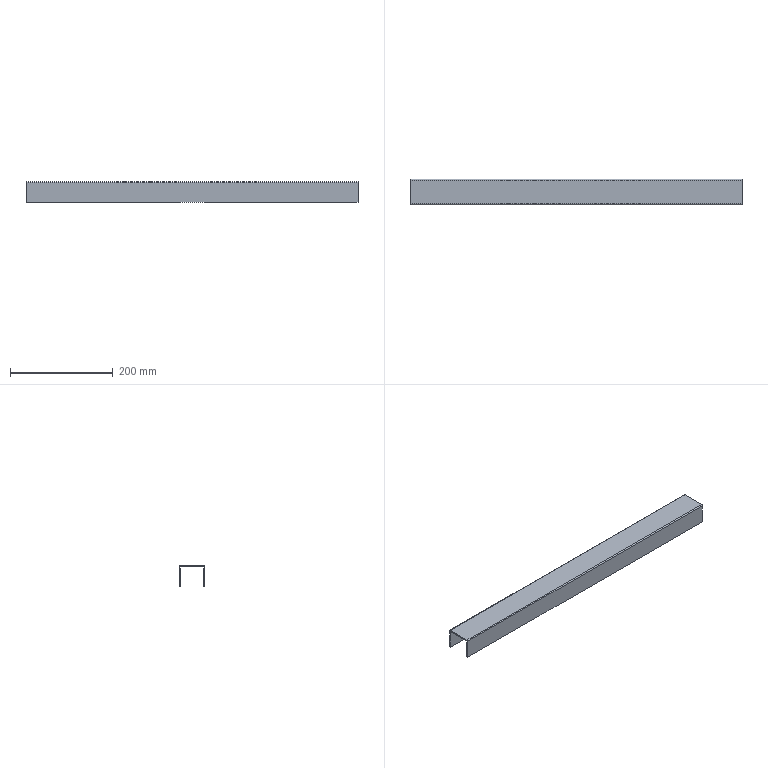Component | SolidWorks | FrameAssembly-1_FrameWeldment-1_LowerBendPlate-1 | 1 solid | 24 faces | box 645 x 50 x 40 mm | volume 195847 mm3 | plane 18 | cylinder 6 | commonest cylinder face diameters 9 x4 4 x2
build123d program:
from build123d import *

# Parameters (mm, degrees)
BOSS_EXTRUDE1_DEPTH = 645
SKETCH6_W           = 37.5
SKETCH6_H           = 45
CUT_EXTRUDE1_DEPTH  = 649.171
CUT_EXTRUDE2_REACH  = 330.795
SKETCH7_W           = 30
SKETCH7_H           = 50
CUT_EXTRUDE3_DEPTH  = 329.424
CUT_EXTRUDE4_REACH  = 330.795


with BuildPart() as part:
    # Sketch5 → Boss-Extrude1 (new body)
    with BuildSketch(Plane(origin=(0, 0, -322.5), x_dir=(-1, 0, 0), z_dir=(0, 0, -1))):
        with BuildLine():
            Line((-40, 50), (-40, 0))
            Line((-40, 0), (-2, 0))
            ThreePointArc((-2, 0), (-0.5858, 0.5858), (0, 2))
            Line((0, 2), (0, 48))
            ThreePointArc((0, 48), (-0.5858, 49.414), (-2, 50))
            Line((-2, 50), (-40, 50))
        make_face()
    extrude(amount=-BOSS_EXTRUDE1_DEPTH)

    # Sketch6 → Cut-Extrude1 (cut, through all)
    with BuildSketch(Plane.XY.offset(322.5)):
        with Locations((21.25, 25)):
            Rectangle(SKETCH6_W, SKETCH6_H)
    extrude(amount=-CUT_EXTRUDE1_DEPTH, mode=Mode.SUBTRACT)

    # Sketch7 → Cut-Extrude2 (cut, up to next)
    with BuildSketch(Plane.XZ, mode=Mode.PRIVATE) as cut_extrude2_sk1:
        with Locations((25, 0)):
            Rectangle(SKETCH7_W, SKETCH7_H)
    cut_extrude2_tool1 = extrude(cut_extrude2_sk1.sketch, amount=-CUT_EXTRUDE2_REACH, mode=Mode.PRIVATE) & part.part
    add(cut_extrude2_tool1.solids().sort_by_distance((25, 0, 0))[0], mode=Mode.SUBTRACT)

    # Sketch8 → Cut-Extrude3 (cut, through all)
    with BuildSketch(Plane(origin=(0, 2.5, 0), x_dir=(-1, 0, 0), z_dir=(0, 1, 0))):
        with BuildLine():
            Line((-26, -247.5), (-14, -247.5))
            ThreePointArc((-14, -247.5), (-9.5, -243), (-14, -238.5))
            Line((-14, -238.5), (-26, -238.5))
            ThreePointArc((-26, -238.5), (-30.5, -243), (-26, -247.5))
        make_face()
    extrude(amount=-CUT_EXTRUDE3_DEPTH, mode=Mode.SUBTRACT)

    # Sketch9 → Cut-Extrude4 (cut, up to next)
    with BuildSketch(Plane.XZ, mode=Mode.PRIVATE) as cut_extrude4_sk1:
        with BuildLine():
            Line((26, 247.5), (14, 247.5))
            ThreePointArc((14, 247.5), (9.5, 243), (14, 238.5))
            Line((14, 238.5), (26, 238.5))
            ThreePointArc((26, 238.5), (30.5, 243), (26, 247.5))
        make_face()
    cut_extrude4_tool1 = extrude(cut_extrude4_sk1.sketch, amount=-CUT_EXTRUDE4_REACH, mode=Mode.PRIVATE) & part.part
    add(cut_extrude4_tool1.solids().sort_by_distance((20, 0, 243))[0], mode=Mode.SUBTRACT)


solid = part.part

# Placed as in the assembly
solid = solid.moved(Location((-298.746, -158.627, -16.5), (180, -90, 0)))
STEP:
#1=COLOUR_RGB('',0.7922,0.8196,0.9333);
#2=FILL_AREA_STYLE_COLOUR('',#1);
#3=FILL_AREA_STYLE('',(#2));
#4=SURFACE_STYLE_FILL_AREA(#3);
#5=SURFACE_SIDE_STYLE('',(#4));
#6=SURFACE_STYLE_USAGE(.BOTH.,#5);
#7=PRESENTATION_STYLE_ASSIGNMENT((#6));
#8=CARTESIAN_POINT('',(-10.777,-6.344,-2.224));
#9=VERTEX_POINT('',#8);
#10=CARTESIAN_POINT('',(-10.777,-6.245,-2.224));
#11=VERTEX_POINT('',#10);
#12=CARTESIAN_POINT('',(-10.777,-8.214,-2.224));
#13=DIRECTION('',(0.,1.,0.));
#14=VECTOR('',#13,39.37);
#15=LINE('',#12,#14);
#16=EDGE_CURVE('',#9,#11,#15,.T.);
#17=ORIENTED_EDGE('',*,*,#16,.T.);
#18=CARTESIAN_POINT('',(0.9352,-6.245,-2.224));
#19=VERTEX_POINT('',#18);
#20=CARTESIAN_POINT('',(-24.459,-6.245,-2.224));
#21=DIRECTION('',(1.,0.,-0.));
#22=VECTOR('',#21,39.37);
#23=LINE('',#20,#22);
#24=EDGE_CURVE('',#11,#19,#23,.T.);
#25=ORIENTED_EDGE('',*,*,#24,.T.);
#26=CARTESIAN_POINT('',(0.9352,-6.344,-2.224));
#27=VERTEX_POINT('',#26);
#28=CARTESIAN_POINT('',(0.9352,-8.214,-2.224));
#29=DIRECTION('',(0.,1.,0.));
#30=VECTOR('',#29,39.37);
#31=LINE('',#28,#30);
#32=EDGE_CURVE('',#27,#19,#31,.T.);
#33=ORIENTED_EDGE('',*,*,#32,.F.);
#34=CARTESIAN_POINT('',(0.9352,-6.344,-2.224));
#35=DIRECTION('',(-1.,0.,0.));
#36=VECTOR('',#35,39.37);
#37=LINE('',#34,#36);
#38=EDGE_CURVE('',#27,#9,#37,.T.);
#39=ORIENTED_EDGE('',*,*,#38,.T.);
#40=EDGE_LOOP('',(#17,#25,#33,#39));
#41=FACE_OUTER_BOUND('',#40,.T.);
#42=CARTESIAN_POINT('',(-24.459,-8.214,-2.224));
#43=DIRECTION('',(-0.,0.,-1.));
#44=DIRECTION('',(1.,0.,-0.));
#45=AXIS2_PLACEMENT_3D('',#42,#43,#44);
#46=PLANE('',#45);
#47=ADVANCED_FACE('',(#41),#46,.T.);
#48=CARTESIAN_POINT('',(-12.746,-6.344,-2.224));
#49=VERTEX_POINT('',#48);
#50=CARTESIAN_POINT('',(-12.746,-6.245,-2.224));
#51=VERTEX_POINT('',#50);
#52=CARTESIAN_POINT('',(-12.746,-8.214,-2.224));
#53=DIRECTION('',(0.,1.,0.));
#54=VECTOR('',#53,39.37);
#55=LINE('',#52,#54);
#56=EDGE_CURVE('',#49,#51,#55,.T.);
#57=ORIENTED_EDGE('',*,*,#56,.F.);
#58=CARTESIAN_POINT('',(-24.459,-6.344,-2.224));
#59=VERTEX_POINT('',#58);
#60=CARTESIAN_POINT('',(0.9352,-6.344,-2.224));
#61=DIRECTION('',(-1.,0.,0.));
#62=VECTOR('',#61,39.37);
#63=LINE('',#60,#62);
#64=EDGE_CURVE('',#49,#59,#63,.T.);
#65=ORIENTED_EDGE('',*,*,#64,.T.);
#66=CARTESIAN_POINT('',(-24.459,-6.245,-2.224));
#67=VERTEX_POINT('',#66);
#68=CARTESIAN_POINT('',(-24.459,-8.214,-2.224));
#69=DIRECTION('',(0.,1.,0.));
#70=VECTOR('',#69,39.37);
#71=LINE('',#68,#70);
#72=EDGE_CURVE('',#59,#67,#71,.T.);
#73=ORIENTED_EDGE('',*,*,#72,.T.);
#74=CARTESIAN_POINT('',(-24.459,-6.245,-2.224));
#75=DIRECTION('',(1.,0.,-0.));
#76=VECTOR('',#75,39.37);
#77=LINE('',#74,#76);
#78=EDGE_CURVE('',#67,#51,#77,.T.);
#79=ORIENTED_EDGE('',*,*,#78,.T.);
#80=EDGE_LOOP('',(#57,#65,#73,#79));
#81=FACE_OUTER_BOUND('',#80,.T.);
#82=CARTESIAN_POINT('',(-24.459,-8.214,-2.224));
#83=DIRECTION('',(-0.,0.,-1.));
#84=DIRECTION('',(1.,0.,-0.));
#85=AXIS2_PLACEMENT_3D('',#82,#83,#84);
#86=PLANE('',#85);
#87=ADVANCED_FACE('',(#81),#86,.T.);
#88=CARTESIAN_POINT('',(0.9352,-8.214,-0.7283));
#89=VERTEX_POINT('',#88);
#90=CARTESIAN_POINT('',(0.9352,-8.214,-2.224));
#91=VERTEX_POINT('',#90);
#92=CARTESIAN_POINT('',(0.9352,-8.214,-0.7283));
#93=DIRECTION('',(-0.,0.,-1.));
#94=VECTOR('',#93,39.37);
#95=LINE('',#92,#94);
#96=EDGE_CURVE('',#89,#91,#95,.T.);
#97=ORIENTED_EDGE('',*,*,#96,.F.);
#98=CARTESIAN_POINT('',(-24.459,-8.214,-0.7283));
#99=VERTEX_POINT('',#98);
#100=CARTESIAN_POINT('',(-24.459,-8.214,-0.7283));
#101=DIRECTION('',(1.,0.,-0.));
#102=VECTOR('',#101,39.37);
#103=LINE('',#100,#102);
#104=EDGE_CURVE('',#99,#89,#103,.T.);
#105=ORIENTED_EDGE('',*,*,#104,.F.);
#106=CARTESIAN_POINT('',(-24.459,-8.214,-2.224));
#107=VERTEX_POINT('',#106);
#108=CARTESIAN_POINT('',(-24.459,-8.214,-0.7283));
#109=DIRECTION('',(-0.,0.,-1.));
#110=VECTOR('',#109,39.37);
#111=LINE('',#108,#110);
#112=EDGE_CURVE('',#99,#107,#111,.T.);
#113=ORIENTED_EDGE('',*,*,#112,.T.);
#114=CARTESIAN_POINT('',(-24.459,-8.214,-2.224));
#115=DIRECTION('',(1.,0.,-0.));
#116=VECTOR('',#115,39.37);
#117=LINE('',#114,#116);
#118=EDGE_CURVE('',#107,#91,#117,.T.);
#119=ORIENTED_EDGE('',*,*,#118,.T.);
#120=EDGE_LOOP('',(#97,#105,#113,#119));
#121=FACE_OUTER_BOUND('',#120,.T.);
#122=CARTESIAN_POINT('',(-24.459,-8.214,-0.7283));
#123=DIRECTION('',(0.,-1.,0.));
#124=DIRECTION('',(-1.,0.,0.));
#125=AXIS2_PLACEMENT_3D('',#122,#123,#124);
#126=PLANE('',#125);
#127=ADVANCED_FACE('',(#121),#126,.T.);
#128=CARTESIAN_POINT('',(0.9352,-8.135,-0.6496));
#129=VERTEX_POINT('',#128);
#130=CARTESIAN_POINT('',(0.9352,-8.135,-0.7283));
#131=DIRECTION('',(1.,0.,-0.));
#132=DIRECTION('',(0.,0.,1.));
#133=AXIS2_PLACEMENT_3D('',#130,#131,#132);
#134=CIRCLE('',#133,0.07874);
#135=EDGE_CURVE('',#129,#89,#134,.T.);
#136=ORIENTED_EDGE('',*,*,#135,.F.);
#137=CARTESIAN_POINT('',(-24.459,-8.135,-0.6496));
#138=VERTEX_POINT('',#137);
#139=CARTESIAN_POINT('',(-24.459,-8.135,-0.6496));
#140=DIRECTION('',(1.,0.,-0.));
#141=VECTOR('',#140,39.37);
#142=LINE('',#139,#141);
#143=EDGE_CURVE('',#138,#129,#142,.T.);
#144=ORIENTED_EDGE('',*,*,#143,.F.);
#145=CARTESIAN_POINT('',(-24.459,-8.135,-0.7283));
#146=DIRECTION('',(1.,0.,-0.));
#147=DIRECTION('',(0.,0.,1.));
#148=AXIS2_PLACEMENT_3D('',#145,#146,#147);
#149=CIRCLE('',#148,0.07874);
#150=EDGE_CURVE('',#138,#99,#149,.T.);
#151=ORIENTED_EDGE('',*,*,#150,.T.);
#152=ORIENTED_EDGE('',*,*,#104,.T.);
#153=EDGE_LOOP('',(#136,#144,#151,#152));
#154=FACE_OUTER_BOUND('',#153,.T.);
#155=CARTESIAN_POINT('',(-24.459,-8.135,-0.7283));
#156=DIRECTION('',(1.,0.,-0.));
#157=DIRECTION('',(0.,0.,1.));
#158=AXIS2_PLACEMENT_3D('',#155,#156,#157);
#159=CYLINDRICAL_SURFACE('',#158,0.07874);
#160=ADVANCED_FACE('',(#154),#159,.T.);
#161=CARTESIAN_POINT('',(0.9352,-6.324,-0.6496));
#162=VERTEX_POINT('',#161);
#163=CARTESIAN_POINT('',(0.9352,-6.324,-0.6496));
#164=DIRECTION('',(0.,-1.,0.));
#165=VECTOR('',#164,39.37);
#166=LINE('',#163,#165);
#167=EDGE_CURVE('',#162,#129,#166,.T.);
#168=ORIENTED_EDGE('',*,*,#167,.F.);
#169=CARTESIAN_POINT('',(-24.459,-6.324,-0.6496));
#170=VERTEX_POINT('',#169);
#171=CARTESIAN_POINT('',(-24.459,-6.324,-0.6496));
#172=DIRECTION('',(1.,0.,-0.));
#173=VECTOR('',#172,39.37);
#174=LINE('',#171,#173);
#175=EDGE_CURVE('',#170,#162,#174,.T.);
#176=ORIENTED_EDGE('',*,*,#175,.F.);
#177=CARTESIAN_POINT('',(-24.459,-6.324,-0.6496));
#178=DIRECTION('',(0.,-1.,0.));
#179=VECTOR('',#178,39.37);
#180=LINE('',#177,#179);
#181=EDGE_CURVE('',#170,#138,#180,.T.);
#182=ORIENTED_EDGE('',*,*,#181,.T.);
#183=ORIENTED_EDGE('',*,*,#143,.T.);
#184=EDGE_LOOP('',(#168,#176,#182,#183));
#185=FACE_OUTER_BOUND('',#184,.T.);
#186=CARTESIAN_POINT('',(-24.459,-6.324,-0.6496));
#187=DIRECTION('',(0.,0.,1.));
#188=DIRECTION('',(-0.,1.,-0.));
#189=AXIS2_PLACEMENT_3D('',#186,#187,#188);
#190=PLANE('',#189);
#191=ADVANCED_FACE('',(#185),#190,.T.);
#192=CARTESIAN_POINT('',(0.9352,-6.245,-0.7283));
#193=VERTEX_POINT('',#192);
#194=CARTESIAN_POINT('',(0.9352,-6.324,-0.7283));
#195=DIRECTION('',(1.,0.,-0.));
#196=DIRECTION('',(0.,0.,1.));
#197=AXIS2_PLACEMENT_3D('',#194,#195,#196);
#198=CIRCLE('',#197,0.07874);
#199=EDGE_CURVE('',#193,#162,#198,.T.);
#200=ORIENTED_EDGE('',*,*,#199,.F.);
#201=CARTESIAN_POINT('',(-24.459,-6.245,-0.7283));
#202=VERTEX_POINT('',#201);
#203=CARTESIAN_POINT('',(-24.459,-6.245,-0.7283));
#204=DIRECTION('',(1.,0.,-0.));
#205=VECTOR('',#204,39.37);
#206=LINE('',#203,#205);
#207=EDGE_CURVE('',#202,#193,#206,.T.);
#208=ORIENTED_EDGE('',*,*,#207,.F.);
#209=CARTESIAN_POINT('',(-24.459,-6.324,-0.7283));
#210=DIRECTION('',(1.,0.,-0.));
#211=DIRECTION('',(0.,0.,1.));
#212=AXIS2_PLACEMENT_3D('',#209,#210,#211);
#213=CIRCLE('',#212,0.07874);
#214=EDGE_CURVE('',#202,#170,#213,.T.);
#215=ORIENTED_EDGE('',*,*,#214,.T.);
#216=ORIENTED_EDGE('',*,*,#175,.T.);
#217=EDGE_LOOP('',(#200,#208,#215,#216));
#218=FACE_OUTER_BOUND('',#217,.T.);
#219=CARTESIAN_POINT('',(-24.459,-6.324,-0.7283));
#220=DIRECTION('',(1.,0.,-0.));
#221=DIRECTION('',(0.,0.,1.));
#222=AXIS2_PLACEMENT_3D('',#219,#220,#221);
#223=CYLINDRICAL_SURFACE('',#222,0.07874);
#224=ADVANCED_FACE('',(#218),#223,.T.);
#225=CARTESIAN_POINT('',(-21.151,-6.245,-1.673));
#226=VERTEX_POINT('',#225);
#227=CARTESIAN_POINT('',(-21.506,-6.245,-1.673));
#228=VERTEX_POINT('',#227);
#229=CARTESIAN_POINT('',(-21.329,-6.245,-1.673));
#230=DIRECTION('',(0.,1.,0.));
#231=DIRECTION('',(1.,0.,0.));
#232=AXIS2_PLACEMENT_3D('',#229,#230,#231);
#233=CIRCLE('',#232,0.1772);
#234=EDGE_CURVE('',#226,#228,#233,.T.);
#235=ORIENTED_EDGE('',*,*,#234,.F.);
#236=CARTESIAN_POINT('',(-21.151,-6.245,-1.201));
#237=VERTEX_POINT('',#236);
#238=CARTESIAN_POINT('',(-21.151,-6.245,-1.201));
#239=DIRECTION('',(0.,0.,-1.));
#240=VECTOR('',#239,39.37);
#241=LINE('',#238,#240);
#242=EDGE_CURVE('',#237,#226,#241,.T.);
#243=ORIENTED_EDGE('',*,*,#242,.F.);
#244=CARTESIAN_POINT('',(-21.506,-6.245,-1.201));
#245=VERTEX_POINT('',#244);
#246=CARTESIAN_POINT('',(-21.329,-6.245,-1.201));
#247=DIRECTION('',(0.,1.,0.));
#248=DIRECTION('',(1.,0.,0.));
#249=AXIS2_PLACEMENT_3D('',#246,#247,#248);
#250=CIRCLE('',#249,0.1772);
#251=EDGE_CURVE('',#245,#237,#250,.T.);
#252=ORIENTED_EDGE('',*,*,#251,.F.);
#253=CARTESIAN_POINT('',(-21.506,-6.245,-1.673));
#254=DIRECTION('',(0.,0.,1.));
#255=VECTOR('',#254,39.37);
#256=LINE('',#253,#255);
#257=EDGE_CURVE('',#228,#245,#256,.T.);
#258=ORIENTED_EDGE('',*,*,#257,.F.);
#259=EDGE_LOOP('',(#235,#243,#252,#258));
#260=FACE_BOUND('',#259,.T.);
#261=CARTESIAN_POINT('',(-2.372,-6.245,-1.673));
#262=VERTEX_POINT('',#261);
#263=CARTESIAN_POINT('',(-2.018,-6.245,-1.673));
#264=VERTEX_POINT('',#263);
#265=CARTESIAN_POINT('',(-2.195,-6.245,-1.673));
#266=DIRECTION('',(0.,-1.,0.));
#267=DIRECTION('',(-1.,0.,0.));
#268=AXIS2_PLACEMENT_3D('',#265,#266,#267);
#269=CIRCLE('',#268,0.1772);
#270=EDGE_CURVE('',#262,#264,#269,.T.);
#271=ORIENTED_EDGE('',*,*,#270,.T.);
#272=CARTESIAN_POINT('',(-2.018,-6.245,-1.201));
#273=VERTEX_POINT('',#272);
#274=CARTESIAN_POINT('',(-2.018,-6.245,-1.673));
#275=DIRECTION('',(0.,0.,1.));
#276=VECTOR('',#275,39.37);
#277=LINE('',#274,#276);
#278=EDGE_CURVE('',#264,#273,#277,.T.);
#279=ORIENTED_EDGE('',*,*,#278,.T.);
#280=CARTESIAN_POINT('',(-2.372,-6.245,-1.201));
#281=VERTEX_POINT('',#280);
#282=CARTESIAN_POINT('',(-2.195,-6.245,-1.201));
#283=DIRECTION('',(0.,-1.,0.));
#284=DIRECTION('',(-1.,0.,0.));
#285=AXIS2_PLACEMENT_3D('',#282,#283,#284);
#286=CIRCLE('',#285,0.1772);
#287=EDGE_CURVE('',#273,#281,#286,.T.);
#288=ORIENTED_EDGE('',*,*,#287,.T.);
#289=CARTESIAN_POINT('',(-2.372,-6.245,-1.201));
#290=DIRECTION('',(-0.,0.,-1.));
#291=VECTOR('',#290,39.37);
#292=LINE('',#289,#291);
#293=EDGE_CURVE('',#281,#262,#292,.T.);
#294=ORIENTED_EDGE('',*,*,#293,.T.);
#295=EDGE_LOOP('',(#271,#279,#288,#294));
#296=FACE_BOUND('',#295,.T.);
#297=CARTESIAN_POINT('',(-10.777,-6.245,-1.043));
#298=VERTEX_POINT('',#297);
#299=CARTESIAN_POINT('',(-10.777,-6.245,-1.043));
#300=DIRECTION('',(-0.,0.,-1.));
#301=VECTOR('',#300,39.37);
#302=LINE('',#299,#301);
#303=EDGE_CURVE('',#298,#11,#302,.T.);
#304=ORIENTED_EDGE('',*,*,#303,.F.);
#305=CARTESIAN_POINT('',(-12.746,-6.245,-1.043));
#306=VERTEX_POINT('',#305);
#307=CARTESIAN_POINT('',(-12.746,-6.245,-1.043));
#308=DIRECTION('',(1.,0.,-0.));
#309=VECTOR('',#308,39.37);
#310=LINE('',#307,#309);
#311=EDGE_CURVE('',#306,#298,#310,.T.);
#312=ORIENTED_EDGE('',*,*,#311,.F.);
#313=CARTESIAN_POINT('',(-12.746,-6.245,-2.224));
#314=DIRECTION('',(0.,0.,1.));
#315=VECTOR('',#314,39.37);
#316=LINE('',#313,#315);
#317=EDGE_CURVE('',#51,#306,#316,.T.);
#318=ORIENTED_EDGE('',*,*,#317,.F.);
#319=ORIENTED_EDGE('',*,*,#78,.F.);
#320=CARTESIAN_POINT('',(-24.459,-6.245,-2.224));
#321=DIRECTION('',(0.,0.,1.));
#322=VECTOR('',#321,39.37);
#323=LINE('',#320,#322);
#324=EDGE_CURVE('',#67,#202,#323,.T.);
#325=ORIENTED_EDGE('',*,*,#324,.T.);
#326=ORIENTED_EDGE('',*,*,#207,.T.);
#327=CARTESIAN_POINT('',(0.9352,-6.245,-2.224));
#328=DIRECTION('',(0.,0.,1.));
#329=VECTOR('',#328,39.37);
#330=LINE('',#327,#329);
#331=EDGE_CURVE('',#19,#193,#330,.T.);
#332=ORIENTED_EDGE('',*,*,#331,.F.);
#333=ORIENTED_EDGE('',*,*,#24,.F.);
#334=EDGE_LOOP('',(#304,#312,#318,#319,#325,#326,#332,#333));
#335=FACE_OUTER_BOUND('',#334,.T.);
#336=CARTESIAN_POINT('',(-24.459,-6.245,-2.224));
#337=DIRECTION('',(0.,1.,0.));
#338=DIRECTION('',(1.,0.,-0.));
#339=AXIS2_PLACEMENT_3D('',#336,#337,#338);
#340=PLANE('',#339);
#341=ADVANCED_FACE('',(#260,#296,#335),#340,.T.);
#342=CARTESIAN_POINT('',(0.9352,-8.115,-2.224));
#343=VERTEX_POINT('',#342);
#344=CARTESIAN_POINT('',(-24.459,-8.115,-2.224));
#345=VERTEX_POINT('',#344);
#346=CARTESIAN_POINT('',(0.9352,-8.115,-2.224));
#347=DIRECTION('',(-1.,0.,0.));
#348=VECTOR('',#347,39.37);
#349=LINE('',#346,#348);
#350=EDGE_CURVE('',#343,#345,#349,.T.);
#351=ORIENTED_EDGE('',*,*,#350,.F.);
#352=CARTESIAN_POINT('',(0.9352,-8.214,-2.224));
#353=DIRECTION('',(0.,1.,0.));
#354=VECTOR('',#353,39.37);
#355=LINE('',#352,#354);
#356=EDGE_CURVE('',#91,#343,#355,.T.);
#357=ORIENTED_EDGE('',*,*,#356,.F.);
#358=ORIENTED_EDGE('',*,*,#118,.F.);
#359=CARTESIAN_POINT('',(-24.459,-8.214,-2.224));
#360=DIRECTION('',(0.,1.,0.));
#361=VECTOR('',#360,39.37);
#362=LINE('',#359,#361);
#363=EDGE_CURVE('',#107,#345,#362,.T.);
#364=ORIENTED_EDGE('',*,*,#363,.T.);
#365=EDGE_LOOP('',(#351,#357,#358,#364));
#366=FACE_OUTER_BOUND('',#365,.T.);
#367=CARTESIAN_POINT('',(-24.459,-8.214,-2.224));
#368=DIRECTION('',(-0.,0.,-1.));
#369=DIRECTION('',(1.,0.,-0.));
#370=AXIS2_PLACEMENT_3D('',#367,#368,#369);
#371=PLANE('',#370);
#372=ADVANCED_FACE('',(#366),#371,.T.);
#373=ORIENTED_EDGE('',*,*,#72,.F.);
#374=CARTESIAN_POINT('',(-24.459,-6.344,-0.748));
#375=VERTEX_POINT('',#374);
#376=CARTESIAN_POINT('',(-24.459,-6.344,-0.748));
#377=DIRECTION('',(-0.,0.,-1.));
#378=VECTOR('',#377,39.37);
#379=LINE('',#376,#378);
#380=EDGE_CURVE('',#375,#59,#379,.T.);
#381=ORIENTED_EDGE('',*,*,#380,.F.);
#382=CARTESIAN_POINT('',(-24.459,-8.115,-0.748));
#383=VERTEX_POINT('',#382);
#384=CARTESIAN_POINT('',(-24.459,-8.115,-0.748));
#385=DIRECTION('',(0.,1.,0.));
#386=VECTOR('',#385,39.37);
#387=LINE('',#384,#386);
#388=EDGE_CURVE('',#383,#375,#387,.T.);
#389=ORIENTED_EDGE('',*,*,#388,.F.);
#390=CARTESIAN_POINT('',(-24.459,-8.115,-2.224));
#391=DIRECTION('',(0.,0.,1.));
#392=VECTOR('',#391,39.37);
#393=LINE('',#390,#392);
#394=EDGE_CURVE('',#345,#383,#393,.T.);
#395=ORIENTED_EDGE('',*,*,#394,.F.);
#396=ORIENTED_EDGE('',*,*,#363,.F.);
#397=ORIENTED_EDGE('',*,*,#112,.F.);
#398=ORIENTED_EDGE('',*,*,#150,.F.);
#399=ORIENTED_EDGE('',*,*,#181,.F.);
#400=ORIENTED_EDGE('',*,*,#214,.F.);
#401=ORIENTED_EDGE('',*,*,#324,.F.);
#402=EDGE_LOOP('',(#373,#381,#389,#395,#396,#397,#398,#399,#400,#401));
#403=FACE_OUTER_BOUND('',#402,.T.);
#404=CARTESIAN_POINT('',(-24.459,-6.324,-0.7283));
#405=DIRECTION('',(1.,0.,-0.));
#406=DIRECTION('',(0.,0.,1.));
#407=AXIS2_PLACEMENT_3D('',#404,#405,#406);
#408=PLANE('',#407);
#409=ADVANCED_FACE('',(#403),#408,.F.);
#410=CARTESIAN_POINT('',(0.9352,-6.344,-0.748));
#411=VERTEX_POINT('',#410);
#412=CARTESIAN_POINT('',(0.9352,-6.344,-0.748));
#413=DIRECTION('',(-0.,0.,-1.));
#414=VECTOR('',#413,39.37);
#415=LINE('',#412,#414);
#416=EDGE_CURVE('',#411,#27,#415,.T.);
#417=ORIENTED_EDGE('',*,*,#416,.T.);
#418=ORIENTED_EDGE('',*,*,#32,.T.);
#419=ORIENTED_EDGE('',*,*,#331,.T.);
#420=ORIENTED_EDGE('',*,*,#199,.T.);
#421=ORIENTED_EDGE('',*,*,#167,.T.);
#422=ORIENTED_EDGE('',*,*,#135,.T.);
#423=ORIENTED_EDGE('',*,*,#96,.T.);
#424=ORIENTED_EDGE('',*,*,#356,.T.);
#425=CARTESIAN_POINT('',(0.9352,-8.115,-0.748));
#426=VERTEX_POINT('',#425);
#427=CARTESIAN_POINT('',(0.9352,-8.115,-2.224));
#428=DIRECTION('',(0.,0.,1.));
#429=VECTOR('',#428,39.37);
#430=LINE('',#427,#429);
#431=EDGE_CURVE('',#343,#426,#430,.T.);
#432=ORIENTED_EDGE('',*,*,#431,.T.);
#433=CARTESIAN_POINT('',(0.9352,-8.115,-0.748));
#434=DIRECTION('',(0.,1.,0.));
#435=VECTOR('',#434,39.37);
#436=LINE('',#433,#435);
#437=EDGE_CURVE('',#426,#411,#436,.T.);
#438=ORIENTED_EDGE('',*,*,#437,.T.);
#439=EDGE_LOOP('',(#417,#418,#419,#420,#421,#422,#423,#424,#432,#438));
#440=FACE_OUTER_BOUND('',#439,.T.);
#441=CARTESIAN_POINT('',(0.9352,-6.324,-0.7283));
#442=DIRECTION('',(1.,0.,-0.));
#443=DIRECTION('',(0.,0.,1.));
#444=AXIS2_PLACEMENT_3D('',#441,#442,#443);
#445=PLANE('',#444);
#446=ADVANCED_FACE('',(#440),#445,.T.);
#447=CARTESIAN_POINT('',(-21.151,-6.344,-1.673));
#448=VERTEX_POINT('',#447);
#449=CARTESIAN_POINT('',(-21.151,-6.344,-1.201));
#450=VERTEX_POINT('',#449);
#451=CARTESIAN_POINT('',(-21.151,-6.344,-1.201));
#452=DIRECTION('',(-0.,0.,1.));
#453=VECTOR('',#452,39.37);
#454=LINE('',#451,#453);
#455=EDGE_CURVE('',#448,#450,#454,.T.);
#456=ORIENTED_EDGE('',*,*,#455,.F.);
#457=CARTESIAN_POINT('',(-21.506,-6.344,-1.673));
#458=VERTEX_POINT('',#457);
#459=CARTESIAN_POINT('',(-21.329,-6.344,-1.673));
#460=DIRECTION('',(0.,-1.,0.));
#461=DIRECTION('',(1.,0.,0.));
#462=AXIS2_PLACEMENT_3D('',#459,#460,#461);
#463=CIRCLE('',#462,0.1772);
#464=EDGE_CURVE('',#458,#448,#463,.T.);
#465=ORIENTED_EDGE('',*,*,#464,.F.);
#466=CARTESIAN_POINT('',(-21.506,-6.344,-1.201));
#467=VERTEX_POINT('',#466);
#468=CARTESIAN_POINT('',(-21.506,-6.344,-1.673));
#469=DIRECTION('',(-0.,0.,-1.));
#470=VECTOR('',#469,39.37);
#471=LINE('',#468,#470);
#472=EDGE_CURVE('',#467,#458,#471,.T.);
#473=ORIENTED_EDGE('',*,*,#472,.F.);
#474=CARTESIAN_POINT('',(-21.329,-6.344,-1.201));
#475=DIRECTION('',(0.,-1.,0.));
#476=DIRECTION('',(1.,0.,0.));
#477=AXIS2_PLACEMENT_3D('',#474,#475,#476);
#478=CIRCLE('',#477,0.1772);
#479=EDGE_CURVE('',#450,#467,#478,.T.);
#480=ORIENTED_EDGE('',*,*,#479,.F.);
#481=EDGE_LOOP('',(#456,#465,#473,#480));
#482=FACE_BOUND('',#481,.T.);
#483=CARTESIAN_POINT('',(-2.018,-6.344,-1.673));
#484=VERTEX_POINT('',#483);
#485=CARTESIAN_POINT('',(-2.018,-6.344,-1.201));
#486=VERTEX_POINT('',#485);
#487=CARTESIAN_POINT('',(-2.018,-6.344,-1.673));
#488=DIRECTION('',(0.,0.,1.));
#489=VECTOR('',#488,39.37);
#490=LINE('',#487,#489);
#491=EDGE_CURVE('',#484,#486,#490,.T.);
#492=ORIENTED_EDGE('',*,*,#491,.F.);
#493=CARTESIAN_POINT('',(-2.372,-6.344,-1.673));
#494=VERTEX_POINT('',#493);
#495=CARTESIAN_POINT('',(-2.195,-6.344,-1.673));
#496=DIRECTION('',(0.,-1.,0.));
#497=DIRECTION('',(-1.,0.,0.));
#498=AXIS2_PLACEMENT_3D('',#495,#496,#497);
#499=CIRCLE('',#498,0.1772);
#500=EDGE_CURVE('',#494,#484,#499,.T.);
#501=ORIENTED_EDGE('',*,*,#500,.F.);
#502=CARTESIAN_POINT('',(-2.372,-6.344,-1.201));
#503=VERTEX_POINT('',#502);
#504=CARTESIAN_POINT('',(-2.372,-6.344,-1.201));
#505=DIRECTION('',(-0.,0.,-1.));
#506=VECTOR('',#505,39.37);
#507=LINE('',#504,#506);
#508=EDGE_CURVE('',#503,#494,#507,.T.);
#509=ORIENTED_EDGE('',*,*,#508,.F.);
#510=CARTESIAN_POINT('',(-2.195,-6.344,-1.201));
#511=DIRECTION('',(0.,-1.,0.));
#512=DIRECTION('',(-1.,0.,0.));
#513=AXIS2_PLACEMENT_3D('',#510,#511,#512);
#514=CIRCLE('',#513,0.1772);
#515=EDGE_CURVE('',#486,#503,#514,.T.);
#516=ORIENTED_EDGE('',*,*,#515,.F.);
#517=EDGE_LOOP('',(#492,#501,#509,#516));
#518=FACE_BOUND('',#517,.T.);
#519=CARTESIAN_POINT('',(-10.777,-6.344,-1.043));
#520=VERTEX_POINT('',#519);
#521=CARTESIAN_POINT('',(-12.746,-6.344,-1.043));
#522=VERTEX_POINT('',#521);
#523=CARTESIAN_POINT('',(-12.746,-6.344,-1.043));
#524=DIRECTION('',(-1.,0.,0.));
#525=VECTOR('',#524,39.37);
#526=LINE('',#523,#525);
#527=EDGE_CURVE('',#520,#522,#526,.T.);
#528=ORIENTED_EDGE('',*,*,#527,.F.);
#529=CARTESIAN_POINT('',(-10.777,-6.344,-1.043));
#530=DIRECTION('',(0.,0.,1.));
#531=VECTOR('',#530,39.37);
#532=LINE('',#529,#531);
#533=EDGE_CURVE('',#9,#520,#532,.T.);
#534=ORIENTED_EDGE('',*,*,#533,.F.);
#535=ORIENTED_EDGE('',*,*,#38,.F.);
#536=ORIENTED_EDGE('',*,*,#416,.F.);
#537=CARTESIAN_POINT('',(0.9352,-6.344,-0.748));
#538=DIRECTION('',(-1.,0.,0.));
#539=VECTOR('',#538,39.37);
#540=LINE('',#537,#539);
#541=EDGE_CURVE('',#411,#375,#540,.T.);
#542=ORIENTED_EDGE('',*,*,#541,.T.);
#543=ORIENTED_EDGE('',*,*,#380,.T.);
#544=ORIENTED_EDGE('',*,*,#64,.F.);
#545=CARTESIAN_POINT('',(-12.746,-6.344,-2.224));
#546=DIRECTION('',(-0.,0.,-1.));
#547=VECTOR('',#546,39.37);
#548=LINE('',#545,#547);
#549=EDGE_CURVE('',#522,#49,#548,.T.);
#550=ORIENTED_EDGE('',*,*,#549,.F.);
#551=EDGE_LOOP('',(#528,#534,#535,#536,#542,#543,#544,#550));
#552=FACE_OUTER_BOUND('',#551,.T.);
#553=CARTESIAN_POINT('',(0.9352,-6.344,-0.748));
#554=DIRECTION('',(0.,1.,0.));
#555=DIRECTION('',(1.,0.,-0.));
#556=AXIS2_PLACEMENT_3D('',#553,#554,#555);
#557=PLANE('',#556);
#558=ADVANCED_FACE('',(#482,#518,#552),#557,.F.);
#559=ORIENTED_EDGE('',*,*,#388,.T.);
#560=ORIENTED_EDGE('',*,*,#541,.F.);
#561=ORIENTED_EDGE('',*,*,#437,.F.);
#562=CARTESIAN_POINT('',(0.9352,-8.115,-0.748));
#563=DIRECTION('',(-1.,0.,0.));
#564=VECTOR('',#563,39.37);
#565=LINE('',#562,#564);
#566=EDGE_CURVE('',#426,#383,#565,.T.);
#567=ORIENTED_EDGE('',*,*,#566,.T.);
#568=EDGE_LOOP('',(#559,#560,#561,#567));
#569=FACE_OUTER_BOUND('',#568,.T.);
#570=CARTESIAN_POINT('',(0.9352,-8.115,-0.748));
#571=DIRECTION('',(0.,0.,1.));
#572=DIRECTION('',(-1.,0.,0.));
#573=AXIS2_PLACEMENT_3D('',#570,#571,#572);
#574=PLANE('',#573);
#575=ADVANCED_FACE('',(#569),#574,.F.);
#576=ORIENTED_EDGE('',*,*,#394,.T.);
#577=ORIENTED_EDGE('',*,*,#566,.F.);
#578=ORIENTED_EDGE('',*,*,#431,.F.);
#579=ORIENTED_EDGE('',*,*,#350,.T.);
#580=EDGE_LOOP('',(#576,#577,#578,#579));
#581=FACE_OUTER_BOUND('',#580,.T.);
#582=CARTESIAN_POINT('',(0.9352,-8.115,-2.224));
#583=DIRECTION('',(0.,-1.,0.));
#584=DIRECTION('',(0.,0.,1.));
#585=AXIS2_PLACEMENT_3D('',#582,#583,#584);
#586=PLANE('',#585);
#587=ADVANCED_FACE('',(#581),#586,.F.);
#588=ORIENTED_EDGE('',*,*,#533,.T.);
#589=CARTESIAN_POINT('',(-10.777,-8.214,-1.043));
#590=DIRECTION('',(0.,1.,0.));
#591=VECTOR('',#590,39.37);
#592=LINE('',#589,#591);
#593=EDGE_CURVE('',#520,#298,#592,.T.);
#594=ORIENTED_EDGE('',*,*,#593,.T.);
#595=ORIENTED_EDGE('',*,*,#303,.T.);
#596=ORIENTED_EDGE('',*,*,#16,.F.);
#597=EDGE_LOOP('',(#588,#594,#595,#596));
#598=FACE_OUTER_BOUND('',#597,.T.);
#599=CARTESIAN_POINT('',(-10.777,-8.214,-1.043));
#600=DIRECTION('',(1.,0.,-0.));
#601=DIRECTION('',(0.,0.,1.));
#602=AXIS2_PLACEMENT_3D('',#599,#600,#601);
#603=PLANE('',#602);
#604=ADVANCED_FACE('',(#598),#603,.F.);
#605=ORIENTED_EDGE('',*,*,#527,.T.);
#606=CARTESIAN_POINT('',(-12.746,-8.214,-1.043));
#607=DIRECTION('',(0.,1.,0.));
#608=VECTOR('',#607,39.37);
#609=LINE('',#606,#608);
#610=EDGE_CURVE('',#522,#306,#609,.T.);
#611=ORIENTED_EDGE('',*,*,#610,.T.);
#612=ORIENTED_EDGE('',*,*,#311,.T.);
#613=ORIENTED_EDGE('',*,*,#593,.F.);
#614=EDGE_LOOP('',(#605,#611,#612,#613));
#615=FACE_OUTER_BOUND('',#614,.T.);
#616=CARTESIAN_POINT('',(-12.746,-8.214,-1.043));
#617=DIRECTION('',(0.,0.,1.));
#618=DIRECTION('',(-1.,0.,0.));
#619=AXIS2_PLACEMENT_3D('',#616,#617,#618);
#620=PLANE('',#619);
#621=ADVANCED_FACE('',(#615),#620,.F.);
#622=ORIENTED_EDGE('',*,*,#549,.T.);
#623=ORIENTED_EDGE('',*,*,#56,.T.);
#624=ORIENTED_EDGE('',*,*,#317,.T.);
#625=ORIENTED_EDGE('',*,*,#610,.F.);
#626=EDGE_LOOP('',(#622,#623,#624,#625));
#627=FACE_OUTER_BOUND('',#626,.T.);
#628=CARTESIAN_POINT('',(-12.746,-8.214,-2.224));
#629=DIRECTION('',(-1.,0.,0.));
#630=DIRECTION('',(-0.,0.,-1.));
#631=AXIS2_PLACEMENT_3D('',#628,#629,#630);
#632=PLANE('',#631);
#633=ADVANCED_FACE('',(#627),#632,.F.);
#634=ORIENTED_EDGE('',*,*,#500,.T.);
#635=CARTESIAN_POINT('',(-2.018,-6.245,-1.673));
#636=DIRECTION('',(0.,-1.,0.));
#637=VECTOR('',#636,39.37);
#638=LINE('',#635,#637);
#639=EDGE_CURVE('',#264,#484,#638,.T.);
#640=ORIENTED_EDGE('',*,*,#639,.F.);
#641=ORIENTED_EDGE('',*,*,#270,.F.);
#642=CARTESIAN_POINT('',(-2.372,-6.245,-1.673));
#643=DIRECTION('',(0.,-1.,0.));
#644=VECTOR('',#643,39.37);
#645=LINE('',#642,#644);
#646=EDGE_CURVE('',#262,#494,#645,.T.);
#647=ORIENTED_EDGE('',*,*,#646,.T.);
#648=EDGE_LOOP('',(#634,#640,#641,#647));
#649=FACE_OUTER_BOUND('',#648,.T.);
#650=CARTESIAN_POINT('',(-2.195,-6.245,-1.673));
#651=DIRECTION('',(0.,-1.,0.));
#652=DIRECTION('',(-1.,0.,0.));
#653=AXIS2_PLACEMENT_3D('',#650,#651,#652);
#654=CYLINDRICAL_SURFACE('',#653,0.1772);
#655=ADVANCED_FACE('',(#649),#654,.F.);
#656=ORIENTED_EDGE('',*,*,#508,.T.);
#657=ORIENTED_EDGE('',*,*,#646,.F.);
#658=ORIENTED_EDGE('',*,*,#293,.F.);
#659=CARTESIAN_POINT('',(-2.372,-6.245,-1.201));
#660=DIRECTION('',(0.,-1.,0.));
#661=VECTOR('',#660,39.37);
#662=LINE('',#659,#661);
#663=EDGE_CURVE('',#281,#503,#662,.T.);
#664=ORIENTED_EDGE('',*,*,#663,.T.);
#665=EDGE_LOOP('',(#656,#657,#658,#664));
#666=FACE_OUTER_BOUND('',#665,.T.);
#667=CARTESIAN_POINT('',(-2.372,-6.245,-1.201));
#668=DIRECTION('',(-1.,0.,0.));
#669=DIRECTION('',(-0.,0.,-1.));
#670=AXIS2_PLACEMENT_3D('',#667,#668,#669);
#671=PLANE('',#670);
#672=ADVANCED_FACE('',(#666),#671,.F.);
#673=ORIENTED_EDGE('',*,*,#515,.T.);
#674=ORIENTED_EDGE('',*,*,#663,.F.);
#675=ORIENTED_EDGE('',*,*,#287,.F.);
#676=CARTESIAN_POINT('',(-2.018,-6.245,-1.201));
#677=DIRECTION('',(0.,-1.,0.));
#678=VECTOR('',#677,39.37);
#679=LINE('',#676,#678);
#680=EDGE_CURVE('',#273,#486,#679,.T.);
#681=ORIENTED_EDGE('',*,*,#680,.T.);
#682=EDGE_LOOP('',(#673,#674,#675,#681));
#683=FACE_OUTER_BOUND('',#682,.T.);
#684=CARTESIAN_POINT('',(-2.195,-6.245,-1.201));
#685=DIRECTION('',(0.,-1.,0.));
#686=DIRECTION('',(-1.,0.,0.));
#687=AXIS2_PLACEMENT_3D('',#684,#685,#686);
#688=CYLINDRICAL_SURFACE('',#687,0.1772);
#689=ADVANCED_FACE('',(#683),#688,.F.);
#690=ORIENTED_EDGE('',*,*,#491,.T.);
#691=ORIENTED_EDGE('',*,*,#680,.F.);
#692=ORIENTED_EDGE('',*,*,#278,.F.);
#693=ORIENTED_EDGE('',*,*,#639,.T.);
#694=EDGE_LOOP('',(#690,#691,#692,#693));
#695=FACE_OUTER_BOUND('',#694,.T.);
#696=CARTESIAN_POINT('',(-2.018,-6.245,-1.673));
#697=DIRECTION('',(1.,0.,-0.));
#698=DIRECTION('',(0.,0.,1.));
#699=AXIS2_PLACEMENT_3D('',#696,#697,#698);
#700=PLANE('',#699);
#701=ADVANCED_FACE('',(#695),#700,.F.);
#702=ORIENTED_EDGE('',*,*,#464,.T.);
#703=CARTESIAN_POINT('',(-21.151,-8.214,-1.673));
#704=DIRECTION('',(0.,1.,0.));
#705=VECTOR('',#704,39.37);
#706=LINE('',#703,#705);
#707=EDGE_CURVE('',#448,#226,#706,.T.);
#708=ORIENTED_EDGE('',*,*,#707,.T.);
#709=ORIENTED_EDGE('',*,*,#234,.T.);
#710=CARTESIAN_POINT('',(-21.506,-8.214,-1.673));
#711=DIRECTION('',(0.,1.,0.));
#712=VECTOR('',#711,39.37);
#713=LINE('',#710,#712);
#714=EDGE_CURVE('',#458,#228,#713,.T.);
#715=ORIENTED_EDGE('',*,*,#714,.F.);
#716=EDGE_LOOP('',(#702,#708,#709,#715));
#717=FACE_OUTER_BOUND('',#716,.T.);
#718=CARTESIAN_POINT('',(-21.329,-8.214,-1.673));
#719=DIRECTION('',(0.,1.,0.));
#720=DIRECTION('',(1.,0.,0.));
#721=AXIS2_PLACEMENT_3D('',#718,#719,#720);
#722=CYLINDRICAL_SURFACE('',#721,0.1772);
#723=ADVANCED_FACE('',(#717),#722,.F.);
#724=ORIENTED_EDGE('',*,*,#455,.T.);
#725=CARTESIAN_POINT('',(-21.151,-8.214,-1.201));
#726=DIRECTION('',(0.,1.,0.));
#727=VECTOR('',#726,39.37);
#728=LINE('',#725,#727);
#729=EDGE_CURVE('',#450,#237,#728,.T.);
#730=ORIENTED_EDGE('',*,*,#729,.T.);
#731=ORIENTED_EDGE('',*,*,#242,.T.);
#732=ORIENTED_EDGE('',*,*,#707,.F.);
#733=EDGE_LOOP('',(#724,#730,#731,#732));
#734=FACE_OUTER_BOUND('',#733,.T.);
#735=CARTESIAN_POINT('',(-21.151,-8.214,-1.201));
#736=DIRECTION('',(1.,0.,0.));
#737=DIRECTION('',(-0.,0.,1.));
#738=AXIS2_PLACEMENT_3D('',#735,#736,#737);
#739=PLANE('',#738);
#740=ADVANCED_FACE('',(#734),#739,.F.);
#741=ORIENTED_EDGE('',*,*,#479,.T.);
#742=CARTESIAN_POINT('',(-21.506,-8.214,-1.201));
#743=DIRECTION('',(0.,1.,0.));
#744=VECTOR('',#743,39.37);
#745=LINE('',#742,#744);
#746=EDGE_CURVE('',#467,#245,#745,.T.);
#747=ORIENTED_EDGE('',*,*,#746,.T.);
#748=ORIENTED_EDGE('',*,*,#251,.T.);
#749=ORIENTED_EDGE('',*,*,#729,.F.);
#750=EDGE_LOOP('',(#741,#747,#748,#749));
#751=FACE_OUTER_BOUND('',#750,.T.);
#752=CARTESIAN_POINT('',(-21.329,-8.214,-1.201));
#753=DIRECTION('',(0.,1.,0.));
#754=DIRECTION('',(1.,0.,0.));
#755=AXIS2_PLACEMENT_3D('',#752,#753,#754);
#756=CYLINDRICAL_SURFACE('',#755,0.1772);
#757=ADVANCED_FACE('',(#751),#756,.F.);
#758=ORIENTED_EDGE('',*,*,#472,.T.);
#759=ORIENTED_EDGE('',*,*,#714,.T.);
#760=ORIENTED_EDGE('',*,*,#257,.T.);
#761=ORIENTED_EDGE('',*,*,#746,.F.);
#762=EDGE_LOOP('',(#758,#759,#760,#761));
#763=FACE_OUTER_BOUND('',#762,.T.);
#764=CARTESIAN_POINT('',(-21.506,-8.214,-1.673));
#765=DIRECTION('',(-1.,0.,0.));
#766=DIRECTION('',(-0.,0.,-1.));
#767=AXIS2_PLACEMENT_3D('',#764,#765,#766);
#768=PLANE('',#767);
#769=ADVANCED_FACE('',(#763),#768,.F.);
#770=CLOSED_SHELL('',(#47,#87,#127,#160,#191,#224,#341,#372,#409,#446,#558,#575,#587,#604,#621,#633,#655,#672,#689,#701,#723,#740,#757,#769));
#771=MANIFOLD_SOLID_BREP('',#770);
#772=STYLED_ITEM('',(#7),#771);
#773=(LENGTH_UNIT()NAMED_UNIT(*)SI_UNIT($,.METRE.));
#774=LENGTH_MEASURE_WITH_UNIT(LENGTH_MEASURE(0.0254),#773);
#775=DIMENSIONAL_EXPONENTS(1.,0.,0.,0.,0.,0.,0.);
#776=(CONVERSION_BASED_UNIT('',#774)LENGTH_UNIT()NAMED_UNIT(#775));
#777=UNCERTAINTY_MEASURE_WITH_UNIT(LENGTH_MEASURE(0.00001),#776,'','');
#778=(NAMED_UNIT(*)PLANE_ANGLE_UNIT()SI_UNIT($,.RADIAN.));
#779=(NAMED_UNIT(*)SI_UNIT($,.STERADIAN.)SOLID_ANGLE_UNIT());
#780=(GEOMETRIC_REPRESENTATION_CONTEXT(3)GLOBAL_UNCERTAINTY_ASSIGNED_CONTEXT((#777))GLOBAL_UNIT_ASSIGNED_CONTEXT((#776,#778,#779))REPRESENTATION_CONTEXT('',''));
#781=MECHANICAL_DESIGN_GEOMETRIC_PRESENTATION_REPRESENTATION('',(#772),#780);
#782=PRESENTATION_LAYER_ASSIGNMENT('','',(#772));
#783=CARTESIAN_POINT('',(0.,0.,0.));
#784=DIRECTION('',(0.,0.,1.));
#785=DIRECTION('',(1.,0.,0.));
#786=AXIS2_PLACEMENT_3D('',#783,#784,#785);
#787=(LENGTH_UNIT()NAMED_UNIT(*)SI_UNIT($,.METRE.));
#788=LENGTH_MEASURE_WITH_UNIT(LENGTH_MEASURE(0.0254),#787);
#789=DIMENSIONAL_EXPONENTS(1.,0.,0.,0.,0.,0.,0.);
#790=(CONVERSION_BASED_UNIT('',#788)LENGTH_UNIT()NAMED_UNIT(#789));
#791=UNCERTAINTY_MEASURE_WITH_UNIT(LENGTH_MEASURE(0.00001),#790,'','');
#792=(NAMED_UNIT(*)PLANE_ANGLE_UNIT()SI_UNIT($,.RADIAN.));
#793=(NAMED_UNIT(*)SI_UNIT($,.STERADIAN.)SOLID_ANGLE_UNIT());
#794=(GEOMETRIC_REPRESENTATION_CONTEXT(3)GLOBAL_UNCERTAINTY_ASSIGNED_CONTEXT((#791))GLOBAL_UNIT_ASSIGNED_CONTEXT((#790,#792,#793))REPRESENTATION_CONTEXT('',''));
#795=ADVANCED_BREP_SHAPE_REPRESENTATION('',(#771,#786),#794);